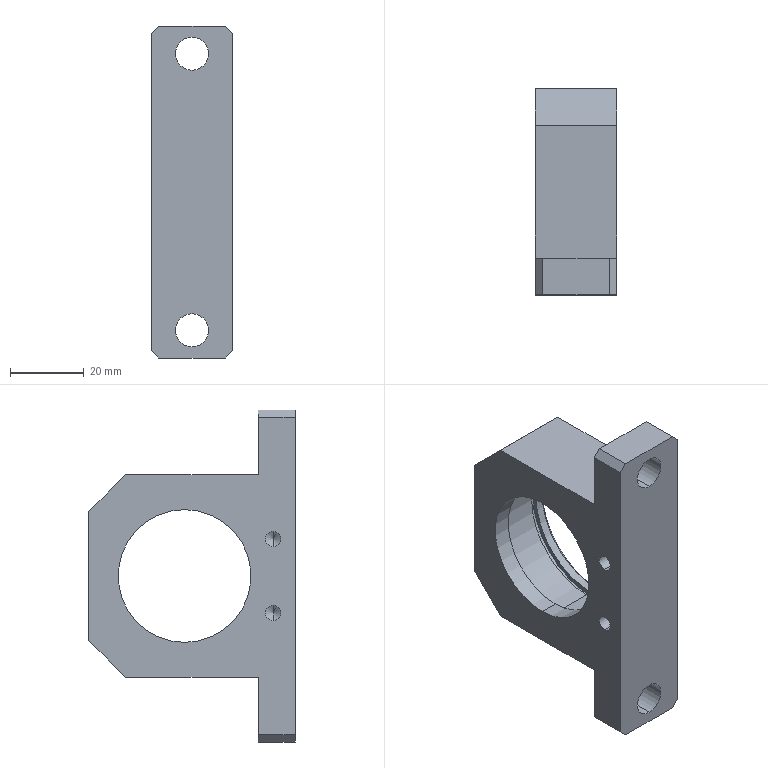Component | SolidWorks | TC020.05-02-3 | 1 solid | 41 faces | volume 42510 mm3 | plane 19 | cylinder 16 | cone 6 | commonest cylinder face diameters 4.2 x4 9 x4 42 x4 44.5 x2 36 x2 | material Q235A